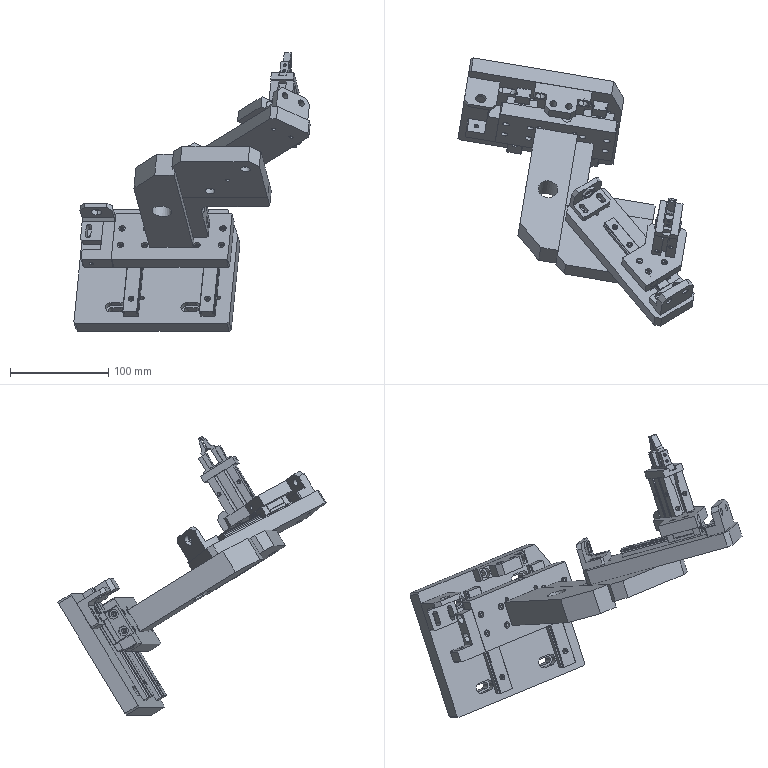Assembly | SolidWorks | mm | 27 component files | 27 solids | 1553 faces | box 240.32 x 272.94 x 283.33 mm | volume 1019614 mm3 | plane 810 | cylinder 445 | cone 149 | spline 145 | torus 4 | commonest cylinder face diameters 3 x44 3.4 x38 4.2 x36 4 x30 2.5 x28 5.5 x28 6.5 x28 10 x24
Bill of materials:
14AC-24-1-001 | 1 |  | Elongated bar or lever. One end is a flat rectangular section with two round through holes. It steps through an angled transition into a tapering arm that ends in a small hooked lip at the tip.
14AC-24-1-002 | 1 |  | Long, flat rectangular plate with chamfered corners. A row of round through holes of mixed sizes runs along its length, and smaller holes appear on one long edge face.
14AC-24-1-003 | 1 |  | L-shaped angle bracket. The base flange has two elongated slots, and the upright flange has one large round through hole. The outer corners are chamfered.
14AC-24-1-004 | 1 |  | Thick plate with an irregular L-shaped or notched outline. The faces carry a pattern of plain and counterbored holes, and a large cross hole runs in from one edge face.
14AC-24-1-005 | 1 |  | Rectangular block or thick plate with a symmetric grid of counterbored and plain holes on its top face, a matching hole pattern on the opposite face, and a side hole on one long edge.
14AC-24-1-006 | 1 |  | Rectangular bar with one large round through hole across its main faces, small holes on a side face and an end face, a narrow step along one long edge, and a chamfered corner at one end.
14AC-24-1-007 | 1 |  | Thick rectangular plate with two chamfered corners at one end. It has three through holes on the main faces (two larger, one smaller between them) and small holes on an end face.
14AC-24-1-008 | 1 |  | Flat L-shaped bracket of rectangular section with a filleted inside corner. It has round holes on its outer faces, two elongated slots through one leg, and two holes on the end face of a leg.
14AC-24-1-009 | 1 |  | Stepped block with an L-shaped profile. The upright portion has two round through holes and the base portion has two more round holes at right angles to them. Some corners are chamfered.
14AC-24-1-010 | 1 |  | L-shaped block (L planform, rectangular section) with small edge chamfers, one hole on the short leg's face, and two holes on the outer side face of the long leg.
14AC-24-1-011 | 1 |  | Elongated block with a stepped (rebated, L-shaped) cross-section along its length. Two round through holes pass through the stepped face.
14AC-24-1-012 | 1 |  | Thick rectangular plate with one chamfered corner. Four counterbored elongated slots sit near the corners, with many small round holes spread across the face and further holes on the edge faces.
14AC-24-1-013 | 1 |  | L-shaped angle bracket with a round hole in one leg and two parallel elongated slots in the other leg; outer corners are chamfered.
14AC-24-1-014 | 1 |  | Rectangular block with a raised central section and lower flanges on each side. Each flange has a counterbored hole, the central section has two through holes, and a hole runs through one end face.
14AC-24-1-015 | 2 |  | Solid round cylinder with flat end faces. One end edge appears slightly rounded or chamfered.
14AC-24-1-016 | 1 |  | Narrow stepped and bent plate. The lower flat section has two round holes, and the upper section is angled and ends in a rounded, hooked lip.
MGN12C | 1 |  | Rectangular block with a channel along its underside. The channel's inner walls have lengthwise grooves. The top face has four holes and a dividing line, separate end-cap segments sit at the ends, and an end face carries engraved lettering and a small hole.
MGN12C-1 | 1 |  | Long straight bar of constant profile with a lengthwise groove in each side. A row of evenly spaced counterbored holes runs through it from the top face.
MGN15C | 2 |  | Rectangular block with a channel along its underside, four holes in the top face, parting lines that separate the end segments, and an end face with a small hole and engraved lettering. The block looks longer than its width.
MGN15C1 | 2 |  | Long straight bar of constant profile with a lengthwise groove in each side and three evenly spaced counterbored through holes from the top face.
MHZ2_16D_Body_0 | 1 |  | Compact rectangular body with lengthwise slots and grooves along its sides. An end plate with a notch is attached to it. One end face has a large circular recess surrounded by several small holes, and the side faces have mounting holes.
MHZ2_16D_Finger_0 | 2 |  | T-shaped block: an upright stem with two round through holes stands on a wider rectangular base. A thin tab or lip sticks out under the base.
SCPG-L-00-16-45-T0H-D-7_5 | 1 |  | Thin hexagonal nut with a plain central bore. Both faces have chamfered corners, and the bore entry is chamfered.
Mates:
1. concentric | MGN12C-1 face at (489.902, -260.171, -68.034) dir (0.5985, -0.711, 0.3692) r 1.25 | MGN12C-1-1 face at (468.657, -234.93, -81.141) dir (0.5985, -0.711, 0.3692) r 1.25
2. concentric | MGN12C-1 face at (480.343, -265.916, -63.603) dir (0.5985, -0.711, 0.3692) r 1.25 | MGN12C-1-1 face at (459.098, -240.675, -76.711) dir (0.5985, -0.711, 0.3692) r 1.25
3. coincident | 14AC-24-1-002-1 face at (416.674, -232.847, -101.209) dir (-0.5985, 0.711, -0.3692) | 14AC-24-1-003-1 face at (439.032, -206.199, -86.134) dir (-0.5985, 0.711, -0.3692)
4. width | 14AC-24-1-003-1 face at (457.122, -194.423, -79.235) dir (0.7966, 0.4787, -0.3692) | 14AC-24-1-003-1 face at (429.243, -211.179, -66.313) dir (-0.7966, -0.4787, 0.3692) | 14AC-24-1-002-1 face at (512.427, -346.608, -42.134) dir (-0.7966, -0.4787, 0.3692) | 14AC-24-1-002-1 face at (552.255, -322.672, -60.595) dir (0.7966, 0.4787, -0.3692)
5. coincident | 14AC-24-1-001-1 face at (528.305, -239.936, -1.101) dir (-0.1401, -0.8413, 0.5222) | MHZ2_16D_M9BL_14_9_0-1/MHZ2_16D_Finger_0-1 face at (521.7, -230.896, 11.692) dir (0.1401, 0.8413, -0.5222)
6. width | 14AC-24-1-004-1 face at (501.702, -303.391, -21.426) dir (0.5985, -0.711, 0.3692) | 14AC-24-1-004-1 face at (477.764, -274.951, -36.195) dir (-0.5985, 0.711, -0.3692) | MGN12C-1 face at (484.975, -281.798, -53.891) dir (-0.5985, 0.711, -0.3692) | MGN12C-1 face at (505.741, -306.47, -41.079) dir (0.5985, -0.711, 0.3692)
7. coincident | 14AC-24-1-004-1 face at (519.603, -271.219, -42.657) dir (0.08576, 0.5151, 0.8529) | MHZ2_16D_M9BL_14_9_0-1/MHZ2_16D_Body_0-1 face at (520.918, -259.95, -49.595) dir (-0.08576, -0.5151, -0.8529)
8. coincident | 14AC-24-1-007-1 face at (508.76, -236.086, -108.513) dir (0.9864, -0.1642, 0) | 14AC-24-1-008-1 face at (507.217, -245.357, -123.864) dir (0.9864, -0.1642, 0)
9. concentric | 14AC-24-1-004-1 face at (495.201, -277.855, -36.195) dir (0.08576, 0.5151, 0.8529) r 1.7 | MGN12C-1 face at (494.258, -283.52, -45.577) dir (-0.08576, -0.5151, -0.8529) r 1.5
10. concentric | 14AC-24-1-004-1 face at (520.109, -278.945, -38.041) dir (0.08576, 0.5151, 0.8529) r 1.7 | MGN12C-1 face at (519.166, -284.611, -47.423) dir (-0.08576, -0.5151, -0.8529) r 1.5
11. coincident | 14AC-24-1-002-1 face at (553.541, -314.946, -47.802) dir (0.08576, 0.5151, 0.8529) | 14AC-24-1-009-2 face at (543.173, -308.328, -50.756) dir (-0.08576, -0.5151, -0.8529)
12. concentric | MGN15C-2 face at (386.193, -98.508, -129.443) dir (-0.08576, -0.5151, -0.8529) r 1.5 | MGN15C1-2 face at (384.367, -109.471, -147.596) dir (-0.08576, -0.5151, -0.8529) r 1.5
13. concentric | MGN15C-2 edge at (368.485, -113.53, -158.397) dir (0.08576, 0.5151, 0.8529) r 1.5 | MGN15C1-2 face at (369.571, -107.007, -147.596) dir (-0.08576, -0.5151, -0.8529) r 1.5
14. concentric | MGN15C1-1 face at (462.294, -122.447, -147.596) dir (-0.08576, -0.5151, -0.8529) r 1.5 | MGN15C-1 face at (464.12, -111.483, -129.443) dir (-0.08576, -0.5151, -0.8529) r 1.5
15. concentric | MGN15C1-1 face at (447.498, -119.983, -147.596) dir (-0.08576, -0.5151, -0.8529) r 1.5 | MGN15C-1 edge at (446.412, -126.506, -158.397) dir (0.08576, 0.5151, 0.8529) r 1.5
16. coincident | MGN15C-1 face at (437.817, -126.372, -157.614) dir (0.08576, 0.5151, 0.8529) | MGN15C-2 face at (359.89, -113.396, -157.614) dir (0.08576, 0.5151, 0.8529)
17. parallel | MGN15C1-1 face at (462.504, -121.185, -148.379) dir (0.9864, -0.1642, 0) | MGN15C1-2 face at (370.481, -101.539, -150.99) dir (-0.9864, 0.1642, 0)
18. coincident | MGN15C1-1 face at (447.008, -122.927, -145.769) dir (-0.1401, -0.8413, 0.5222) | MGN15C1-2 face at (369.081, -109.952, -145.769) dir (-0.1401, -0.8413, 0.5222)
19. coincident | 14AC-24-1-002-1 face at (552.255, -322.672, -60.595) dir (-0.08576, -0.5151, -0.8529) | 14AC-24-1-007-1 face at (498.955, -294.975, -71.962) dir (0.08576, 0.5151, 0.8529)
20. coincident | 14AC-24-1-004-1 face at (519.603, -271.219, -42.657) dir (0.08576, 0.5151, 0.8529) | 14AC-24-1-011-1 face at (524.602, -237.824, -63.327) dir (-0.08576, -0.5151, -0.8529)
21. width | 14AC-24-1-004-1 face at (499.382, -267.521, -56.927) dir (-0.9864, 0.1642, 0) | 14AC-24-1-004-1 face at (536.26, -289.575, -50.834) dir (0.9864, -0.1642, 0) | 14AC-24-1-011-1 face at (536.622, -244.784, -73.231) dir (0.9864, -0.1642, 0) | 14AC-24-1-011-1 face at (510.975, -240.513, -73.231) dir (-0.9864, 0.1642, 0)
22. coincident | 14AC-24-1-004-1 face at (542.46, -252.338, -70.429) dir (0.1401, 0.8413, -0.5222) | 14AC-24-1-011-1 face at (510.938, -240.737, -60.195) dir (-0.1401, -0.8413, 0.5222)
23. coincident | MGN15C1-1 face at (454.82, -115.582, -150.99) dir (0.08576, 0.5151, 0.8529) | MGN15C1-2 face at (376.893, -102.607, -150.99) dir (0.08576, 0.5151, 0.8529)
24. concentric | 14AC-24-1-002-1 face at (469.593, -250.836, -78.078) dir (-0.08576, -0.5151, -0.8529) r 2 | 14AC-24-1-007-1 face at (468.306, -258.562, -90.871) dir (-0.08576, -0.5151, -0.8529) r 2
25. concentric | 14AC-24-1-005-1 face at (461.831, -155.673, -155.29) dir (-0.1401, -0.8413, 0.5222) r 3.25 | MGN15C-1 face at (463.862, -143.474, -162.861) dir (0.1401, 0.8413, -0.5222) r 1.5
26. concentric | 14AC-24-1-005-1 face at (460.115, -165.974, -172.347) dir (-0.1401, -0.8413, 0.5222) r 3.25 | MGN15C-1 face at (462.147, -153.776, -179.918) dir (0.1401, 0.8413, -0.5222) r 1.5
27. concentric | 14AC-24-1-005-1 face at (437.17, -151.567, -155.29) dir (-0.1401, -0.8413, 0.5222) r 3.25 | MGN15C-1 face at (439.201, -139.368, -162.861) dir (0.1401, 0.8413, -0.5222) r 1.5
28. parallel | 14AC-24-1-012-1 face at (394.757, -132.313, -194.059) dir (-0.1401, -0.8413, 0.5222) | 14AC-24-1-013-1 face at (334.355, -108.455, -154.588) dir (-0.1401, -0.8413, 0.5222)
29. distance | 14AC-24-1-006-1 face at (367.788, -272.967, -101.377) dir (-0.1401, -0.8413, 0.5222) | 14AC-24-1-007-1 face at (498.955, -294.975, -71.962) dir (-0.1401, -0.8413, 0.5222)
30. concentric | assembly face at (330.413, -132.13, -166.977) dir (0.08576, 0.5151, 0.8529) r 2.5 | 14AC-24-1-010-1 face at (329.007, -140.57, -180.953) dir (0.08576, 0.5151, 0.8529) r 2.1
31. coincident | 14AC-24-1-005-1 face at (352.853, -128.263, -140.365) dir (-0.9864, 0.1642, 0) | 14AC-24-1-010-1 face at (350.237, -143.973, -195.104) dir (0.9864, -0.1642, 0)
32. coincident | 14AC-24-1-005-1 face at (348.136, -156.592, -187.271) dir (-0.08576, -0.5151, -0.8529) | 14AC-24-1-010-1 face at (350.237, -143.973, -195.104) dir (-0.08576, -0.5151, -0.8529)
33. concentric | 14AC-24-1-005-1 face at (352.617, -129.68, -157.074) dir (-0.9864, 0.1642, 0) r 2.1 | 14AC-24-1-010-1 face at (340.78, -127.709, -157.074) dir (-0.9864, 0.1642, 0) r 2.75
34. concentric | 14AC-24-1-012-1 face at (439.488, -107.206, -141.609) dir (-0.1401, -0.8413, 0.5222) r 2.1 | 14AC-24-1-014-1 face at (437.772, -117.512, -135.212) dir (-0.1401, -0.8413, 0.5222) r 5
35. concentric | 14AC-24-1-012-1 face at (396.085, -99.98, -141.609) dir (-0.1401, -0.8413, 0.5222) r 2.1 | 14AC-24-1-014-1 face at (394.369, -110.285, -135.212) dir (-0.1401, -0.8413, 0.5222) r 5
36. parallel | 14AC-24-1-002-1 face at (512.427, -346.608, -42.134) dir (0.5985, -0.711, 0.3692) | 14AC-24-1-009-2 face at (521.219, -302.418, -36.289) dir (-0.5985, 0.711, -0.3692)
37. concentric | 14AC-24-1-002-1 face at (514.889, -318.903, -41.526) dir (0.08576, 0.5151, 0.8529) r 2.1 | 14AC-24-1-009-2 face at (515.661, -314.267, -33.85) dir (0.08576, 0.5151, 0.8529) r 5
38. concentric | 14AC-24-1-005-1 face at (420.449, -136.308, -150.512) dir (0.08576, 0.5151, 0.8529) r 4.5 | 14AC-24-1-015-1 face at (421.05, -132.702, -144.542) dir (-0.08576, -0.5151, -0.8529) r 4.5
39. coincident | 14AC-24-1-005-1 face at (352.853, -128.263, -140.365) dir (0.08576, 0.5151, 0.8529) | 14AC-24-1-015-1 face at (421.05, -132.702, -144.542) dir (0.08576, 0.5151, 0.8529)
40. coincident | 14AC-24-1-004-1 face at (519.603, -271.219, -42.657) dir (0.08576, 0.5151, 0.8529) | MHZ2_16D_M9BL_14_9_0-1/MHZ2_16D_Body_0-1 face at (520.918, -259.95, -49.595) dir (-0.08576, -0.5151, -0.8529)
41. concentric | 14AC-24-1-004-1 face at (525.746, -276.616, -54.085) dir (-0.08576, -0.5151, -0.8529) r 2.25 | MHZ2_16D_M9BL_14_9_0-1/MHZ2_16D_Body_0-1 face at (526.775, -270.435, -43.851) dir (0.08576, 0.5151, 0.8529) r 1.621
42. concentric | 14AC-24-1-004-1 face at (514.031, -255.645, -65.573) dir (-0.08576, -0.5151, -0.8529) r 4 | MHZ2_16D_M9BL_14_9_0-1/MHZ2_16D_Body_0-1 face at (515.06, -249.464, -55.339) dir (0.08576, 0.5151, 0.8529) r 1.621
43. concentric | 14AC-24-1-004-1 face at (505.803, -295.981, -32.763) dir (0.5985, -0.711, 0.3692) r 4.5 | 14AC-24-1-015-2 face at (509.992, -300.958, -30.179) dir (-0.5985, 0.711, -0.3692) r 4.5
44. coincident | 14AC-24-1-004-1 face at (505.803, -295.981, -32.763) dir (0.5985, -0.711, 0.3692) | 14AC-24-1-015-2 face at (505.803, -295.981, -32.763) dir (-0.5985, 0.711, -0.3692)
45. coincident | 14AC-24-1-007-1 face at (508.76, -236.086, -108.513) dir (0.1401, 0.8413, -0.5222) | 14AC-24-1-008-1 face at (507.217, -245.357, -123.864) dir (-0.1401, -0.8413, 0.5222)
46. concentric | MGN15C1-1 face at (446.258, -173.09, -226.789) dir (0.1401, 0.8413, -0.5222) r 3 | 14AC-24-1-012-1 face at (447.659, -164.678, -232.011) dir (-0.1401, -0.8413, 0.5222) r 1.25
47. concentric | MGN15C1-2 face at (371.26, -142.526, -237.706) dir (0.1401, 0.8413, -0.5222) r 1.75 | 14AC-24-1-012-1 face at (369.732, -151.702, -232.011) dir (-0.1401, -0.8413, 0.5222) r 1.25
48. concentric | MGN15C1-2 face at (378.121, -101.321, -169.478) dir (0.1401, 0.8413, -0.5222) r 1.75 | 14AC-24-1-012-1 face at (376.593, -110.497, -163.783) dir (-0.1401, -0.8413, 0.5222) r 1.25
49. coincident | 14AC-24-1-005-1 face at (411.71, -140.084, -171.389) dir (0.1401, 0.8413, -0.5222) | MGN15C-1 face at (468.262, -138.358, -153.437) dir (-0.1401, -0.8413, 0.5222)
50. coincident | MGN15C1-1 face at (463.205, -116.978, -150.99) dir (0.1401, 0.8413, -0.5222) | 14AC-24-1-012-1 face at (394.757, -132.313, -194.059) dir (-0.1401, -0.8413, 0.5222)
51. concentric | 14AC-24-1-002-1 face at (514.274, -301.071, -52.233) dir (0.08576, 0.5151, 0.8529) r 1.25 | MGN12C-1-1 face at (514.96, -296.951, -45.41) dir (0.08576, 0.5151, 0.8529) r 1.7
52. concentric | 14AC-24-1-002-1 face at (499.313, -283.296, -61.464) dir (0.08576, 0.5151, 0.8529) r 1.25 | MGN12C-1-1 face at (498.543, -287.92, -69.12) dir (-0.08576, -0.5151, -0.8529) r 1.75
53. coincident | 14AC-24-1-007-1 face at (497.411, -304.246, -87.314) dir (-0.08576, -0.5151, -0.8529) | 14AC-24-1-008-1 face at (518.143, -179.739, -164.593) dir (-0.08576, -0.5151, -0.8529)
54. coincident | 14AC-24-1-001-1 face at (531.05, -223.454, 26.191) dir (0.9864, -0.1642, 0) | MHZ2_16D_M9BL_14_9_0-1/MHZ2_16D_Finger_0-1 face at (529.272, -234.132, -11.504) dir (0.9864, -0.1642, 0)
55. coincident | MHZ2_16D_M9BL_14_9_0-1/MHZ2_16D_Finger_0-2 face at (531.679, -219.675, 3.912) dir (-0.1401, -0.8413, 0.5222) | 14AC-24-1-016-1 face at (521.515, -225.923, -8.881) dir (0.1401, 0.8413, -0.5222)
56. coincident | MHZ2_16D_M9BL_14_9_0-1/MHZ2_16D_Finger_0-2 face at (530.392, -227.401, -8.881) dir (0.08576, 0.5151, 0.8529) | 14AC-24-1-016-1 face at (521.515, -225.923, -8.881) dir (-0.08576, -0.5151, -0.8529)
57. coincident | 14AC-24-1-001-1 face at (522.172, -221.976, 26.191) dir (-0.9864, 0.1642, 0) | 14AC-24-1-016-1 face at (524.259, -209.441, 18.41) dir (-0.9864, 0.1642, 0)
58. coincident | 14AC-24-1-001-1 face at (528.305, -239.936, -1.101) dir (-0.08576, -0.5151, -0.8529) | MHZ2_16D_M9BL_14_9_0-1/MHZ2_16D_Finger_0-1 face at (520.414, -238.622, -1.101) dir (0.08576, 0.5151, 0.8529)
59. coincident | 14AC-24-1-004-1 face at (518.66, -276.885, -52.038) dir (-0.08576, -0.5151, -0.8529) | MGN12C-1 face at (507.082, -265.267, -57.89) dir (0.08576, 0.5151, 0.8529)
60. coincident | 14AC-24-1-002-1 face at (553.541, -314.946, -47.802) dir (0.08576, 0.5151, 0.8529) | MGN12C-1-1 face at (468.185, -237.763, -85.832) dir (-0.08576, -0.5151, -0.8529)
61. coincident | 14AC-24-1-002-1 face at (553.541, -314.946, -47.802) dir (0.08576, 0.5151, 0.8529) | 14AC-24-1-003-1 face at (426.927, -225.086, -89.34) dir (-0.08576, -0.5151, -0.8529)
62. coincident | 14AC-24-1-006-1 face at (401.932, -204.897, -116.607) dir (0.08576, 0.5151, 0.8529) | 14AC-24-1-008-1 face at (519.686, -170.467, -149.241) dir (0.08576, 0.5151, 0.8529)
63. coincident | 14AC-24-1-006-1 face at (431.816, -150.234, -173.73) dir (0.9864, -0.1642, 0) | 14AC-24-1-007-1 face at (419.983, -221.304, -108.513) dir (-0.9864, 0.1642, 0)
64. concentric | 14AC-24-1-005-1 face at (423.918, -145.919, -178.473) dir (0.1401, 0.8413, -0.5222) r 2.75 | 14AC-24-1-006-1 face at (421.817, -158.538, -170.641) dir (0.1401, 0.8413, -0.5222) r 2.1
65. concentric | 14AC-24-1-005-1 face at (399.643, -133.408, -164.828) dir (0.1401, 0.8413, -0.5222) r 2.75 | 14AC-24-1-006-1 face at (397.542, -146.027, -156.995) dir (0.1401, 0.8413, -0.5222) r 2.1
66. coincident | 14AC-24-1-005-1 face at (409.679, -152.283, -163.818) dir (-0.1401, -0.8413, 0.5222) | 14AC-24-1-006-1 face at (387.399, -155.19, -174.479) dir (0.1401, 0.8413, -0.5222)
67. angle | 14AC-24-1-002-1 face at (512.427, -346.608, -42.134) dir (-0.7966, -0.4787, 0.3692) | 14AC-24-1-007-1 face at (498.955, -294.975, -71.962) dir (-0.1401, -0.8413, 0.5222)
68. distance | assembly face at (329.013, -145.513, -185.004) dir (-0.08576, -0.5151, -0.8529) | 14AC-24-1-010-1 face at (350.237, -143.973, -195.104) dir (-0.08576, -0.5151, -0.8529)
69. coincident | MHZ2_16D_Body_0-1 axis at (80.9, 0, 46.5) dir (-1, 0, 0) | MHZ2_16D_Finger_0-1 axis at (-83.9, 0, 46.5) dir (1, 0, 0)
70. coincident | MHZ2_16D_Body_0-1 axis at (80.9, 0, 46.5) dir (-1, 0, 0) | MHZ2_16D_Finger_0-1 axis at (-83.9, 0, 46.5) dir (1, 0, 0)
71. coincident | MHZ2_16D_Body_0-1 axis at (80.9, 0, 46.5) dir (-1, 0, 0) | MHZ2_16D_Finger_0-1 axis at (-83.9, 0, 46.5) dir (1, 0, 0)
72. angle | MHZ2_16D_Finger_0-1 plane at (-3, 0, 46.5) dir (0, 0, -1) | MHZ2_16D_Body_0-1 plane at (0, 0, 46.5) dir (0, 0, -1)
73. coincident | MHZ2_16D_Body_0-1 axis at (-80.9, 0, 46.5) dir (1, 0, 0) | MHZ2_16D_Finger_0-2 axis at (83.9, 0, 46.5) dir (-1, 0, 0)
74. coincident | MHZ2_16D_Body_0-1 axis at (-80.9, 0, 46.5) dir (1, 0, 0) | MHZ2_16D_Finger_0-2 axis at (83.9, 0, 46.5) dir (-1, 0, 0)
75. coincident | MHZ2_16D_Body_0-1 axis at (-80.9, 0, 46.5) dir (1, 0, 0) | MHZ2_16D_Finger_0-2 axis at (83.9, 0, 46.5) dir (-1, 0, 0)
76. angle | MHZ2_16D_Finger_0-2 plane at (3, 0, 46.5) dir (0, 0, -1) | MHZ2_16D_Body_0-1 plane at (0, 0, 46.5) dir (0, 0, -1)
77. distance | MHZ2_16D_Finger_0-2 face at (-7.45, 4, 67.3) dir (1, 0, 0) | MHZ2_16D_Finger_0-1 face at (7.45, -4, 67.3) dir (-1, 0, 0)
78. width | MHZ2_16D_Body_0-1 face at (-19, 0, 0) dir (-1, 0, 0) | MHZ2_16D_Body_0-1 face at (19, 0, 0) dir (1, 0, 0) | MHZ2_16D_Finger_0-1 face at (12.45, -4, 52.3) dir (1, 0, 0) | MHZ2_16D_Finger_0-2 face at (-12.45, 4, 52.3) dir (-1, 0, 0)